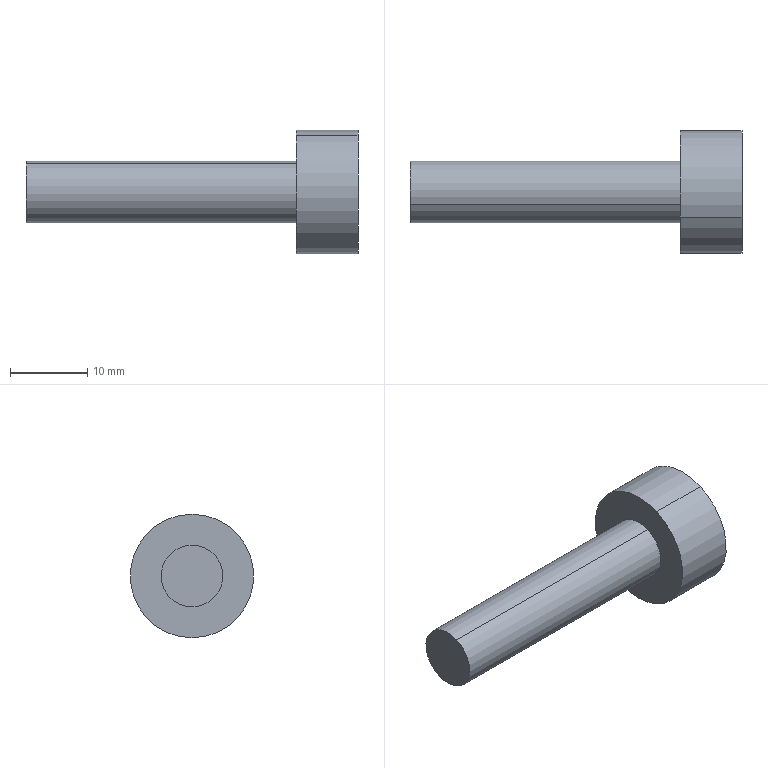Component | SolidWorks | M8Screw-2-1 | 1 solid | 7 faces | box 43 x 16 x 16 mm | volume 3368 mm3 | cylinder 4 | plane 3 | commonest cylinder face diameters 16 x2 8 x2
build123d program:
from build123d import *


with BuildPart() as part:
    # Sketch1 → Revolve1 (revolve)
    with BuildSketch(Plane.XY, mode=Mode.PRIVATE) as revolve1_sk:
        Polygon((0, 0), (0, -43), (4, -43), (4, -8), (8, -8), (8, 0), align=None)
    revolve(revolve1_sk.sketch.rotate(Axis((0, 0, 0), (0, -1, 0)), 180), axis=Axis((0, 0, 0), (0, -1, 0)))


solid = part.part

# Placed as in the assembly
solid = solid.moved(Location((619.036, -118.615, -4.5), (0, 0, -90)))
STEP:
#1=COLOUR_RGB('',0.7922,0.8196,0.9333);
#2=FILL_AREA_STYLE_COLOUR('',#1);
#3=FILL_AREA_STYLE('',(#2));
#4=SURFACE_STYLE_FILL_AREA(#3);
#5=SURFACE_SIDE_STYLE('',(#4));
#6=SURFACE_STYLE_USAGE(.BOTH.,#5);
#7=PRESENTATION_STYLE_ASSIGNMENT((#6));
#8=CARTESIAN_POINT('',(24.057,-4.798,0.1106));
#9=VERTEX_POINT('',#8);
#10=CARTESIAN_POINT('',(24.057,-4.542,-0.4649));
#11=VERTEX_POINT('',#10);
#12=CARTESIAN_POINT('',(24.057,-4.67,-0.1772));
#13=DIRECTION('',(1.,-0.,-0.));
#14=DIRECTION('',(0.,-0.4065,0.9137));
#15=AXIS2_PLACEMENT_3D('',#12,#13,#14);
#16=CIRCLE('',#15,0.315);
#17=EDGE_CURVE('',#9,#11,#16,.T.);
#18=ORIENTED_EDGE('',*,*,#17,.T.);
#19=CARTESIAN_POINT('',(24.372,-4.542,-0.4649));
#20=VERTEX_POINT('',#19);
#21=CARTESIAN_POINT('',(24.372,-4.542,-0.4649));
#22=DIRECTION('',(1.,-0.,-0.));
#23=VECTOR('',#22,39.37);
#24=LINE('',#21,#23);
#25=EDGE_CURVE('',#11,#20,#24,.T.);
#26=ORIENTED_EDGE('',*,*,#25,.T.);
#27=CARTESIAN_POINT('',(24.372,-4.798,0.1106));
#28=VERTEX_POINT('',#27);
#29=CARTESIAN_POINT('',(24.372,-4.67,-0.1772));
#30=DIRECTION('',(1.,-0.,-0.));
#31=DIRECTION('',(0.,-0.4065,0.9137));
#32=AXIS2_PLACEMENT_3D('',#29,#30,#31);
#33=CIRCLE('',#32,0.315);
#34=EDGE_CURVE('',#28,#20,#33,.T.);
#35=ORIENTED_EDGE('',*,*,#34,.F.);
#36=CARTESIAN_POINT('',(24.372,-4.798,0.1106));
#37=DIRECTION('',(1.,-0.,-0.));
#38=VECTOR('',#37,39.37);
#39=LINE('',#36,#38);
#40=EDGE_CURVE('',#9,#28,#39,.T.);
#41=ORIENTED_EDGE('',*,*,#40,.F.);
#42=EDGE_LOOP('',(#18,#26,#35,#41));
#43=FACE_OUTER_BOUND('',#42,.T.);
#44=CARTESIAN_POINT('',(24.372,-4.67,-0.1772));
#45=DIRECTION('',(1.,-0.,-0.));
#46=DIRECTION('',(0.,-0.4065,0.9137));
#47=AXIS2_PLACEMENT_3D('',#44,#45,#46);
#48=CYLINDRICAL_SURFACE('',#47,0.315);
#49=ADVANCED_FACE('',(#43),#48,.T.);
#50=CARTESIAN_POINT('',(22.679,-4.734,-0.03328));
#51=VERTEX_POINT('',#50);
#52=CARTESIAN_POINT('',(22.679,-4.606,-0.321));
#53=VERTEX_POINT('',#52);
#54=CARTESIAN_POINT('',(22.679,-4.67,-0.1772));
#55=DIRECTION('',(1.,-0.,-0.));
#56=DIRECTION('',(0.,-0.4065,0.9137));
#57=AXIS2_PLACEMENT_3D('',#54,#55,#56);
#58=CIRCLE('',#57,0.1575);
#59=EDGE_CURVE('',#51,#53,#58,.T.);
#60=ORIENTED_EDGE('',*,*,#59,.T.);
#61=CARTESIAN_POINT('',(24.057,-4.606,-0.321));
#62=VERTEX_POINT('',#61);
#63=CARTESIAN_POINT('',(24.372,-4.606,-0.321));
#64=DIRECTION('',(1.,-0.,-0.));
#65=VECTOR('',#64,39.37);
#66=LINE('',#63,#65);
#67=EDGE_CURVE('',#53,#62,#66,.T.);
#68=ORIENTED_EDGE('',*,*,#67,.T.);
#69=CARTESIAN_POINT('',(24.057,-4.734,-0.03328));
#70=VERTEX_POINT('',#69);
#71=CARTESIAN_POINT('',(24.057,-4.67,-0.1772));
#72=DIRECTION('',(1.,-0.,-0.));
#73=DIRECTION('',(0.,-0.4065,0.9137));
#74=AXIS2_PLACEMENT_3D('',#71,#72,#73);
#75=CIRCLE('',#74,0.1575);
#76=EDGE_CURVE('',#70,#62,#75,.T.);
#77=ORIENTED_EDGE('',*,*,#76,.F.);
#78=CARTESIAN_POINT('',(24.372,-4.734,-0.03328));
#79=DIRECTION('',(1.,-0.,-0.));
#80=VECTOR('',#79,39.37);
#81=LINE('',#78,#80);
#82=EDGE_CURVE('',#51,#70,#81,.T.);
#83=ORIENTED_EDGE('',*,*,#82,.F.);
#84=EDGE_LOOP('',(#60,#68,#77,#83));
#85=FACE_OUTER_BOUND('',#84,.T.);
#86=CARTESIAN_POINT('',(24.372,-4.67,-0.1772));
#87=DIRECTION('',(1.,-0.,-0.));
#88=DIRECTION('',(0.,-0.4065,0.9137));
#89=AXIS2_PLACEMENT_3D('',#86,#87,#88);
#90=CYLINDRICAL_SURFACE('',#89,0.1575);
#91=ADVANCED_FACE('',(#85),#90,.T.);
#92=ORIENTED_EDGE('',*,*,#34,.T.);
#93=CARTESIAN_POINT('',(24.372,-4.67,-0.1772));
#94=DIRECTION('',(1.,-0.,-0.));
#95=DIRECTION('',(0.,-0.4065,0.9137));
#96=AXIS2_PLACEMENT_3D('',#93,#94,#95);
#97=CIRCLE('',#96,0.315);
#98=EDGE_CURVE('',#20,#28,#97,.T.);
#99=ORIENTED_EDGE('',*,*,#98,.T.);
#100=EDGE_LOOP('',(#92,#99));
#101=FACE_OUTER_BOUND('',#100,.T.);
#102=CARTESIAN_POINT('',(24.372,-4.542,-0.4649));
#103=DIRECTION('',(-1.,0.,0.));
#104=DIRECTION('',(0.,0.4065,-0.9137));
#105=AXIS2_PLACEMENT_3D('',#102,#103,#104);
#106=PLANE('',#105);
#107=ADVANCED_FACE('',(#101),#106,.F.);
#108=ORIENTED_EDGE('',*,*,#59,.F.);
#109=CARTESIAN_POINT('',(22.679,-4.67,-0.1772));
#110=DIRECTION('',(1.,-0.,-0.));
#111=DIRECTION('',(0.,-0.4065,0.9137));
#112=AXIS2_PLACEMENT_3D('',#109,#110,#111);
#113=CIRCLE('',#112,0.1575);
#114=EDGE_CURVE('',#53,#51,#113,.T.);
#115=ORIENTED_EDGE('',*,*,#114,.F.);
#116=EDGE_LOOP('',(#108,#115));
#117=FACE_OUTER_BOUND('',#116,.T.);
#118=CARTESIAN_POINT('',(22.679,-4.67,-0.1772));
#119=DIRECTION('',(1.,-0.,-0.));
#120=DIRECTION('',(-0.,-0.4065,0.9137));
#121=AXIS2_PLACEMENT_3D('',#118,#119,#120);
#122=PLANE('',#121);
#123=ADVANCED_FACE('',(#117),#122,.F.);
#124=ORIENTED_EDGE('',*,*,#67,.F.);
#125=ORIENTED_EDGE('',*,*,#114,.T.);
#126=ORIENTED_EDGE('',*,*,#82,.T.);
#127=CARTESIAN_POINT('',(24.057,-4.67,-0.1772));
#128=DIRECTION('',(1.,-0.,-0.));
#129=DIRECTION('',(0.,-0.4065,0.9137));
#130=AXIS2_PLACEMENT_3D('',#127,#128,#129);
#131=CIRCLE('',#130,0.1575);
#132=EDGE_CURVE('',#62,#70,#131,.T.);
#133=ORIENTED_EDGE('',*,*,#132,.F.);
#134=EDGE_LOOP('',(#124,#125,#126,#133));
#135=FACE_OUTER_BOUND('',#134,.T.);
#136=CARTESIAN_POINT('',(24.372,-4.67,-0.1772));
#137=DIRECTION('',(1.,-0.,-0.));
#138=DIRECTION('',(0.,-0.4065,0.9137));
#139=AXIS2_PLACEMENT_3D('',#136,#137,#138);
#140=CYLINDRICAL_SURFACE('',#139,0.1575);
#141=ADVANCED_FACE('',(#135),#140,.T.);
#142=ORIENTED_EDGE('',*,*,#17,.F.);
#143=CARTESIAN_POINT('',(24.057,-4.67,-0.1772));
#144=DIRECTION('',(1.,-0.,-0.));
#145=DIRECTION('',(0.,-0.4065,0.9137));
#146=AXIS2_PLACEMENT_3D('',#143,#144,#145);
#147=CIRCLE('',#146,0.315);
#148=EDGE_CURVE('',#11,#9,#147,.T.);
#149=ORIENTED_EDGE('',*,*,#148,.F.);
#150=EDGE_LOOP('',(#142,#149));
#151=FACE_OUTER_BOUND('',#150,.T.);
#152=ORIENTED_EDGE('',*,*,#76,.T.);
#153=ORIENTED_EDGE('',*,*,#132,.T.);
#154=EDGE_LOOP('',(#152,#153));
#155=FACE_BOUND('',#154,.T.);
#156=CARTESIAN_POINT('',(24.057,-4.606,-0.321));
#157=DIRECTION('',(1.,-0.,-0.));
#158=DIRECTION('',(-0.,-0.4065,0.9137));
#159=AXIS2_PLACEMENT_3D('',#156,#157,#158);
#160=PLANE('',#159);
#161=ADVANCED_FACE('',(#151,#155),#160,.F.);
#162=ORIENTED_EDGE('',*,*,#25,.F.);
#163=ORIENTED_EDGE('',*,*,#148,.T.);
#164=ORIENTED_EDGE('',*,*,#40,.T.);
#165=ORIENTED_EDGE('',*,*,#98,.F.);
#166=EDGE_LOOP('',(#162,#163,#164,#165));
#167=FACE_OUTER_BOUND('',#166,.T.);
#168=CARTESIAN_POINT('',(24.372,-4.67,-0.1772));
#169=DIRECTION('',(1.,-0.,-0.));
#170=DIRECTION('',(0.,-0.4065,0.9137));
#171=AXIS2_PLACEMENT_3D('',#168,#169,#170);
#172=CYLINDRICAL_SURFACE('',#171,0.315);
#173=ADVANCED_FACE('',(#167),#172,.T.);
#174=CLOSED_SHELL('',(#49,#91,#107,#123,#141,#161,#173));
#175=MANIFOLD_SOLID_BREP('',#174);
#176=STYLED_ITEM('',(#7),#175);
#177=PRESENTATION_LAYER_ASSIGNMENT('','',(#176));
#178=(LENGTH_UNIT()NAMED_UNIT(*)SI_UNIT($,.METRE.));
#179=LENGTH_MEASURE_WITH_UNIT(LENGTH_MEASURE(0.0254),#178);
#180=DIMENSIONAL_EXPONENTS(1.,0.,0.,0.,0.,0.,0.);
#181=(CONVERSION_BASED_UNIT('',#179)LENGTH_UNIT()NAMED_UNIT(#180));
#182=UNCERTAINTY_MEASURE_WITH_UNIT(LENGTH_MEASURE(0.00001),#181,'','');
#183=(NAMED_UNIT(*)PLANE_ANGLE_UNIT()SI_UNIT($,.RADIAN.));
#184=(NAMED_UNIT(*)SI_UNIT($,.STERADIAN.)SOLID_ANGLE_UNIT());
#185=(GEOMETRIC_REPRESENTATION_CONTEXT(3)GLOBAL_UNCERTAINTY_ASSIGNED_CONTEXT((#182))GLOBAL_UNIT_ASSIGNED_CONTEXT((#181,#183,#184))REPRESENTATION_CONTEXT('',''));
#186=MECHANICAL_DESIGN_GEOMETRIC_PRESENTATION_REPRESENTATION('',(#176),#185);
#187=CARTESIAN_POINT('',(0.,0.,0.));
#188=DIRECTION('',(0.,0.,1.));
#189=DIRECTION('',(1.,0.,0.));
#190=AXIS2_PLACEMENT_3D('',#187,#188,#189);
#191=(LENGTH_UNIT()NAMED_UNIT(*)SI_UNIT($,.METRE.));
#192=LENGTH_MEASURE_WITH_UNIT(LENGTH_MEASURE(0.0254),#191);
#193=DIMENSIONAL_EXPONENTS(1.,0.,0.,0.,0.,0.,0.);
#194=(CONVERSION_BASED_UNIT('',#192)LENGTH_UNIT()NAMED_UNIT(#193));
#195=UNCERTAINTY_MEASURE_WITH_UNIT(LENGTH_MEASURE(0.00001),#194,'','');
#196=(NAMED_UNIT(*)PLANE_ANGLE_UNIT()SI_UNIT($,.RADIAN.));
#197=(NAMED_UNIT(*)SI_UNIT($,.STERADIAN.)SOLID_ANGLE_UNIT());
#198=(GEOMETRIC_REPRESENTATION_CONTEXT(3)GLOBAL_UNCERTAINTY_ASSIGNED_CONTEXT((#195))GLOBAL_UNIT_ASSIGNED_CONTEXT((#194,#196,#197))REPRESENTATION_CONTEXT('',''));
#199=ADVANCED_BREP_SHAPE_REPRESENTATION('',(#175,#190),#198);